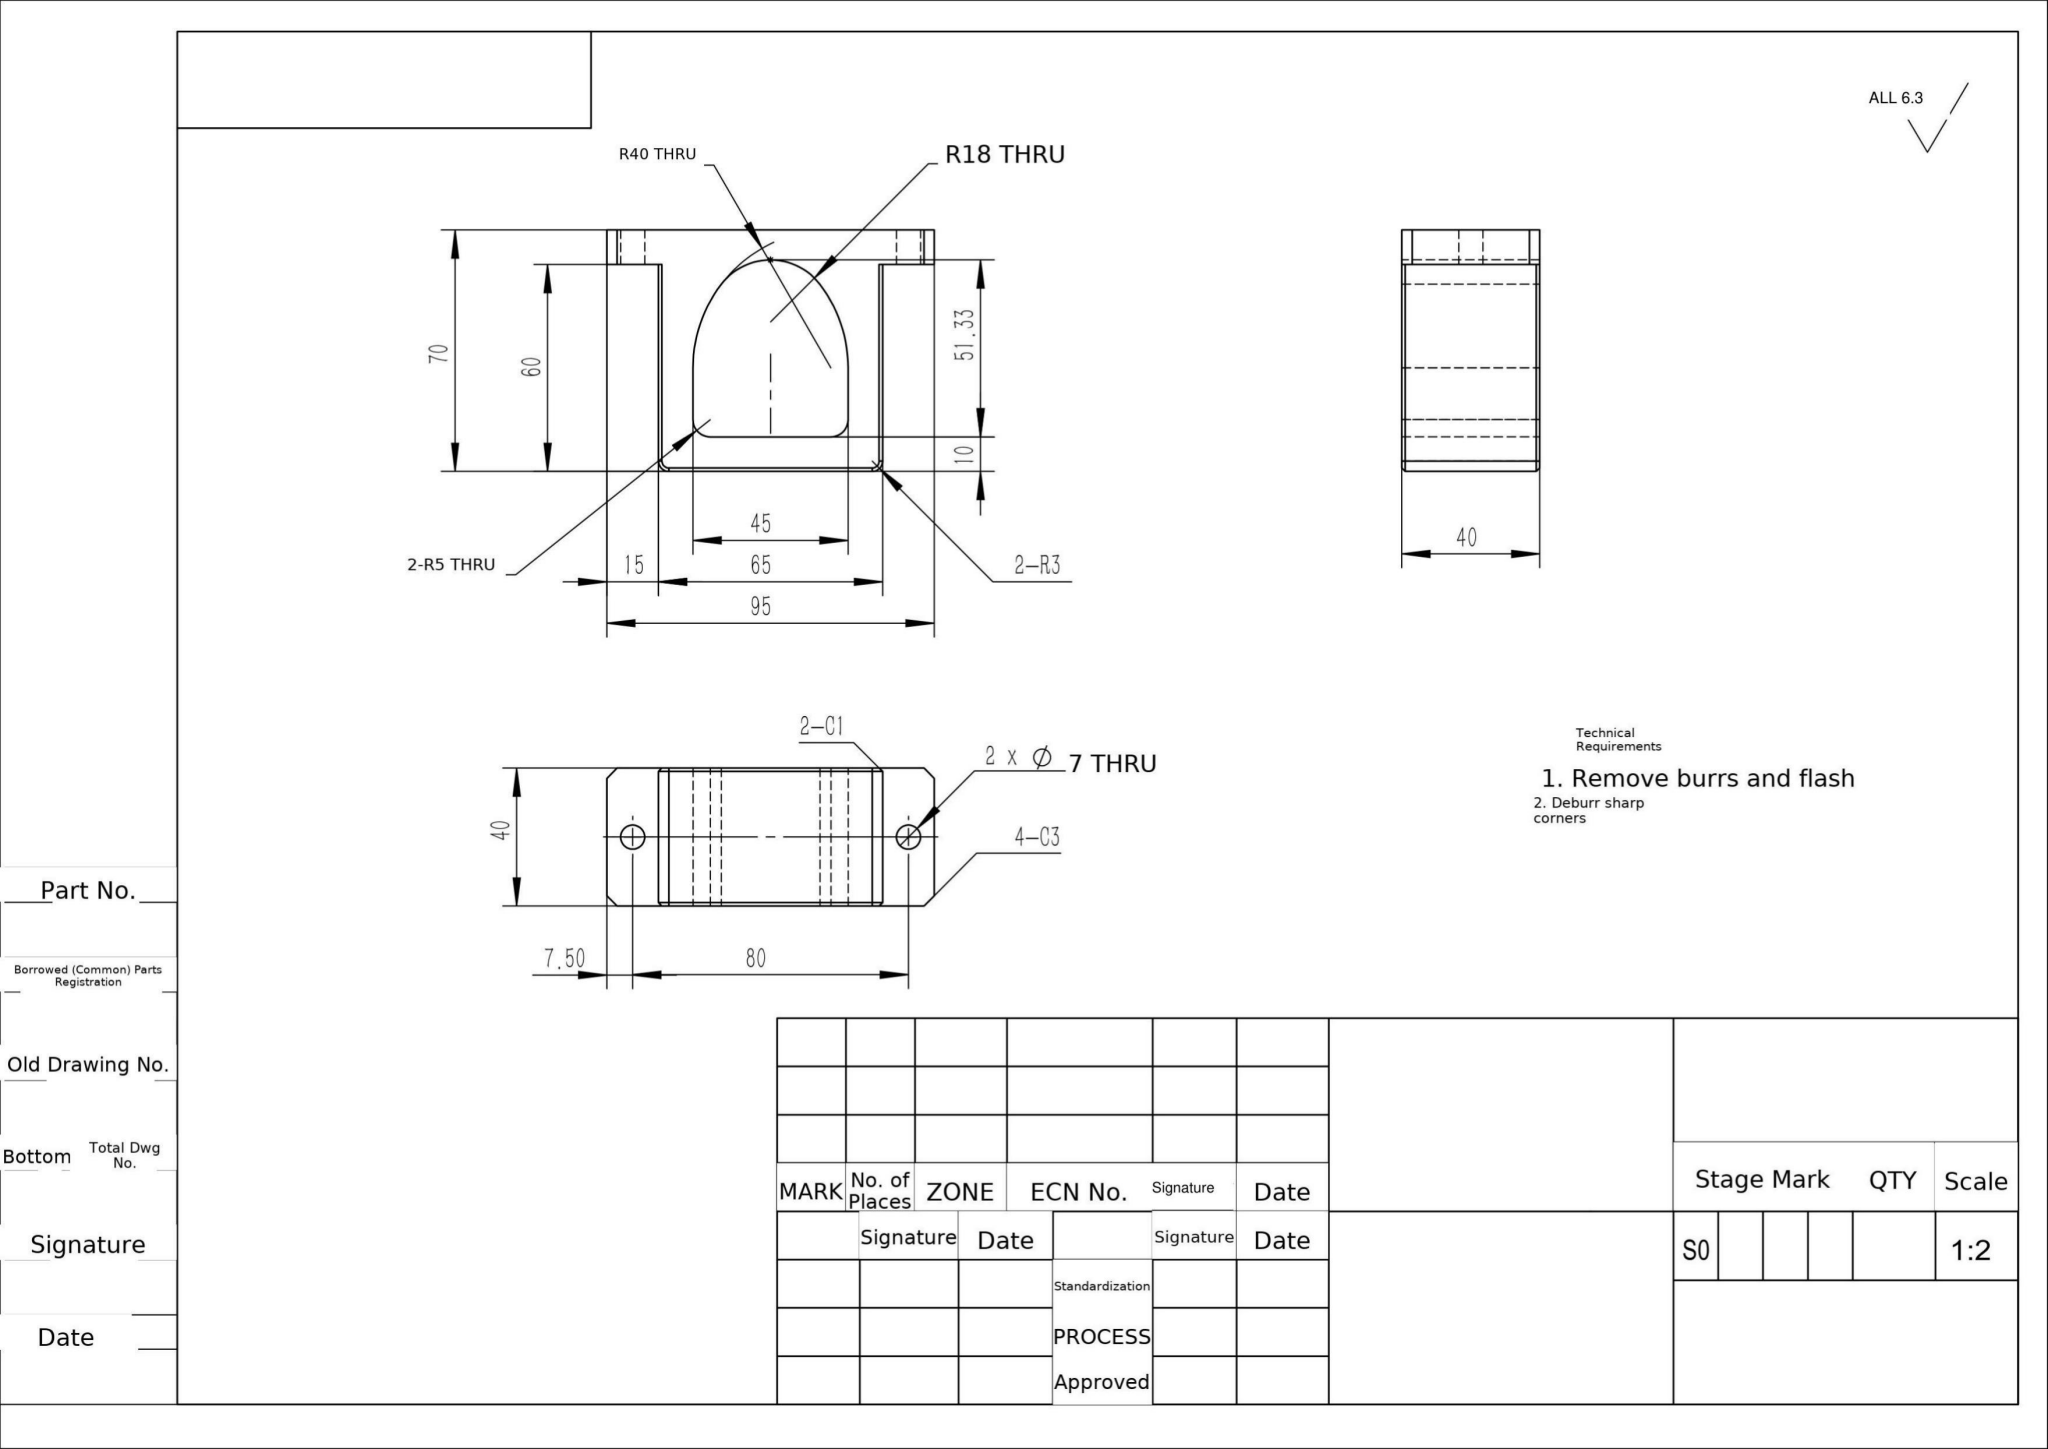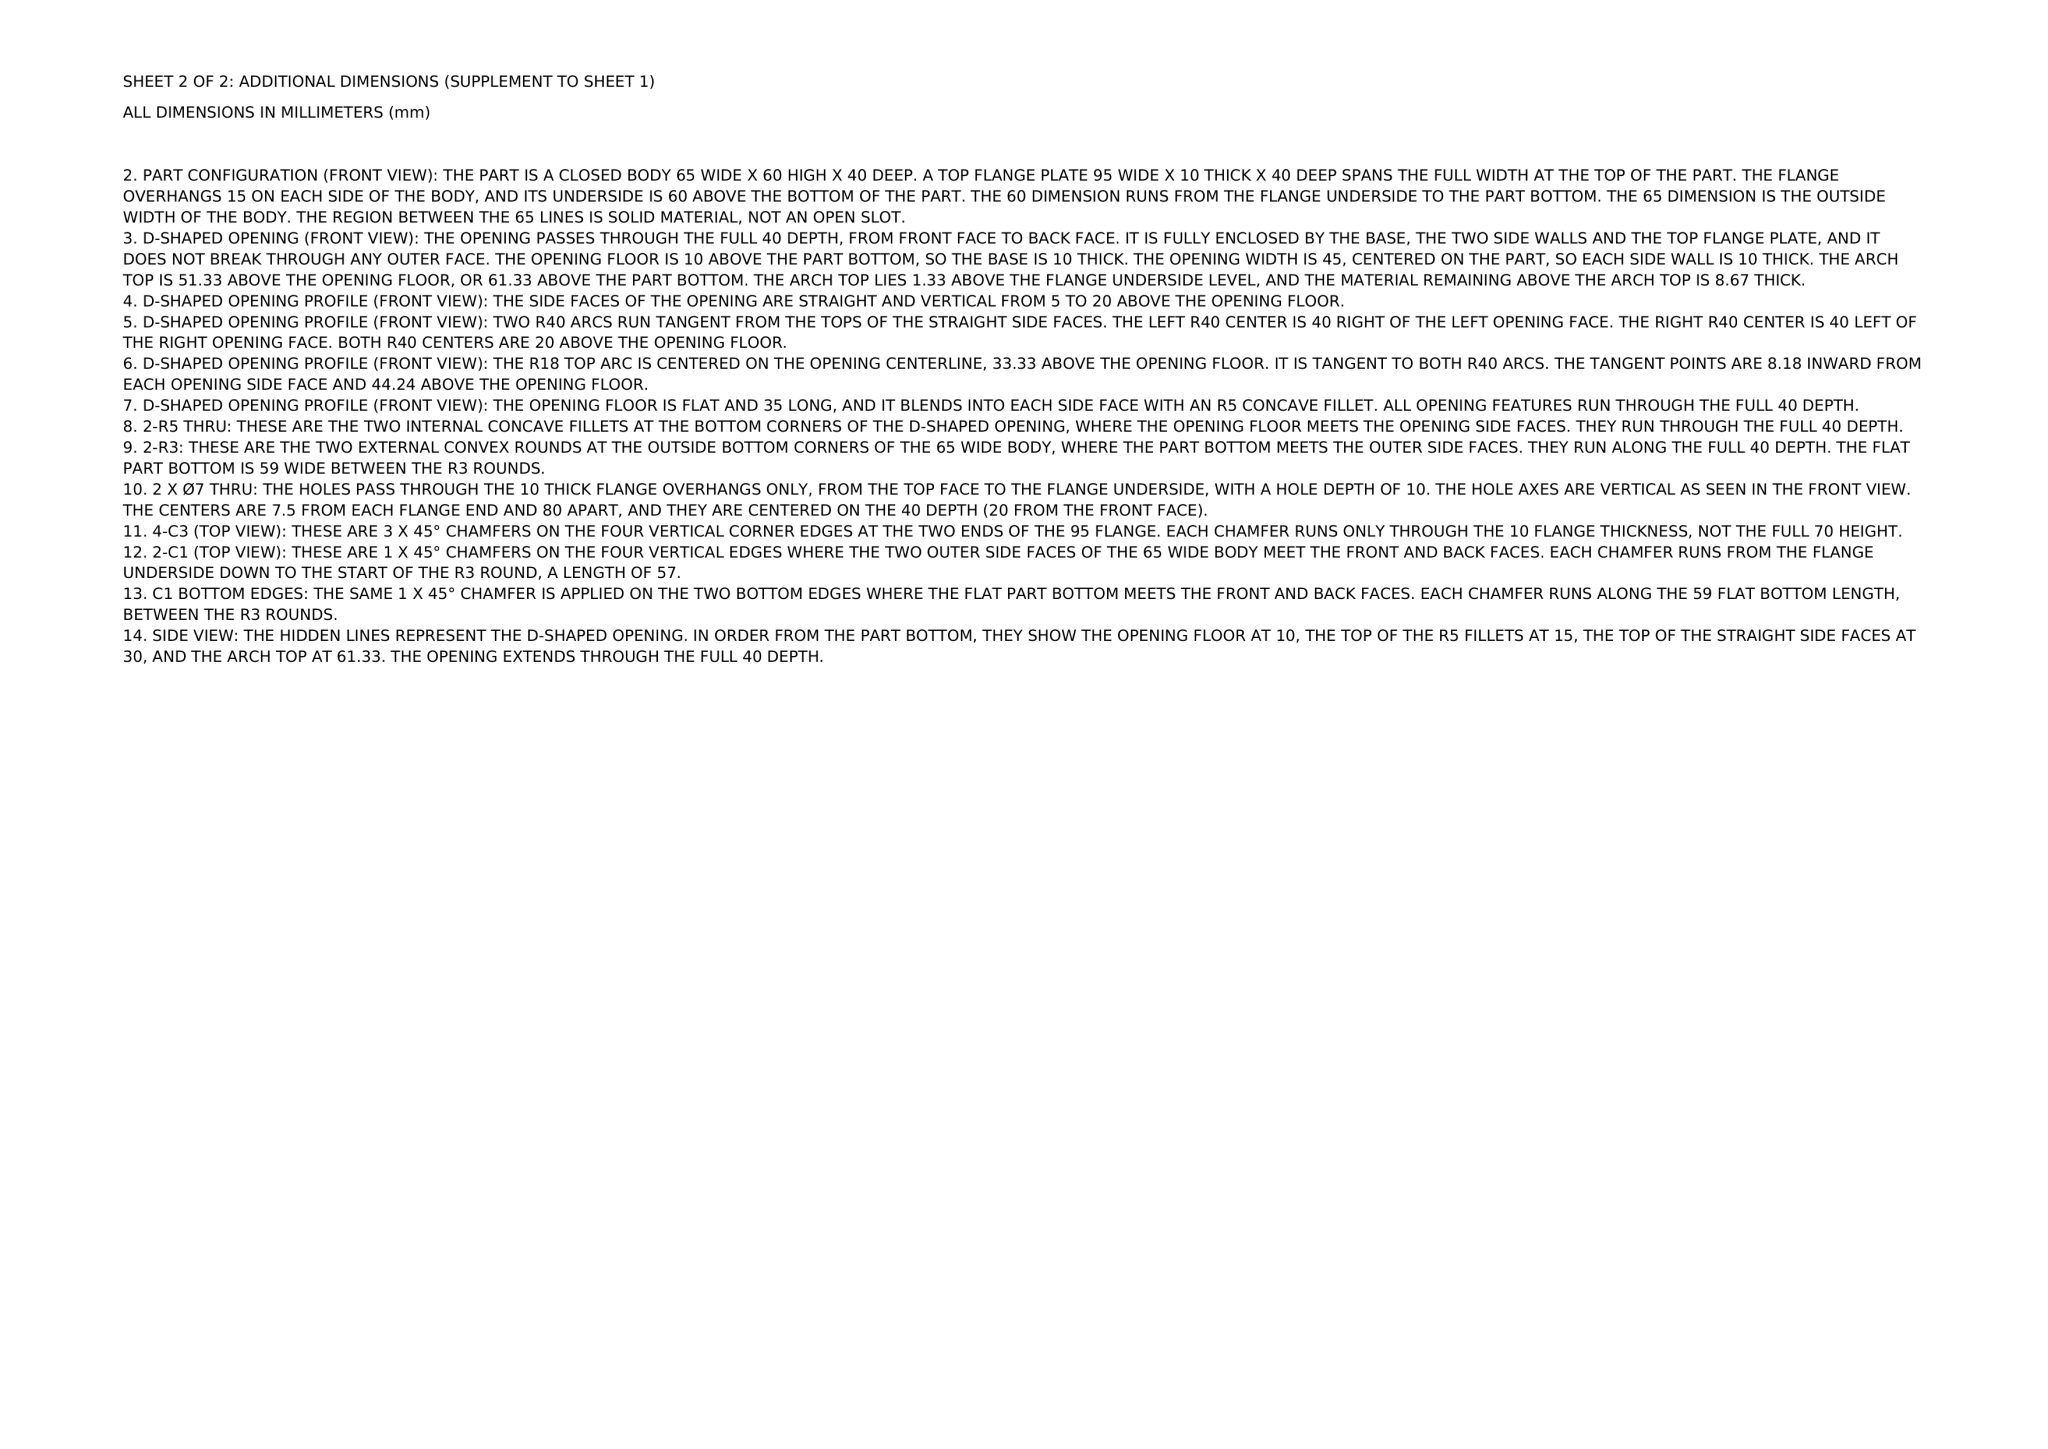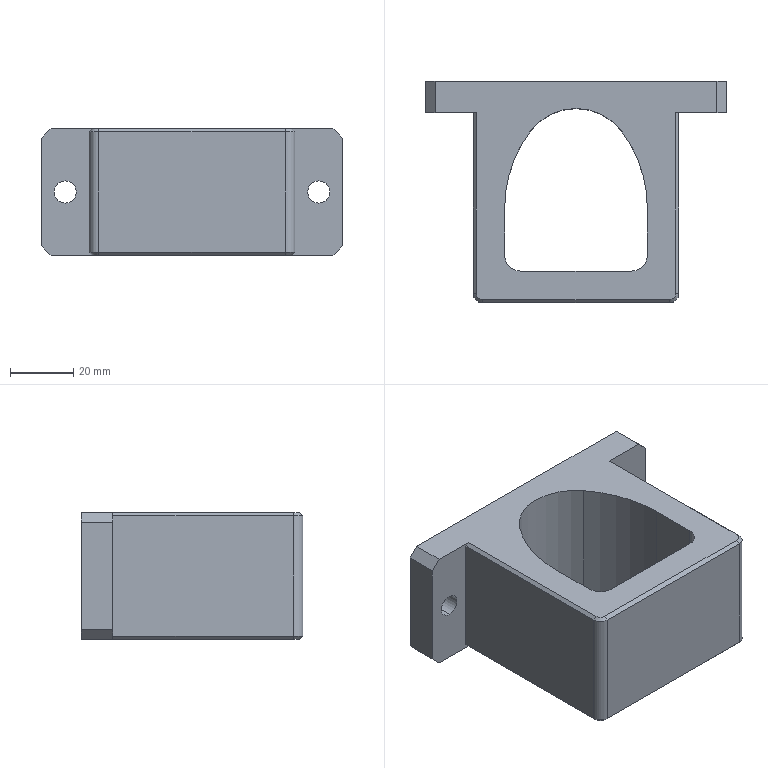Part | NX | mm | Flanged Cavity Mounting Block | 1 solid | 38 faces | box 95 x 70 x 40 mm | volume 112890 mm3 | plane 23 | cylinder 11 | cone 4 | commonest cylinder face diameters 7 x4 80 x2 10 x2 6 x2 36 x1